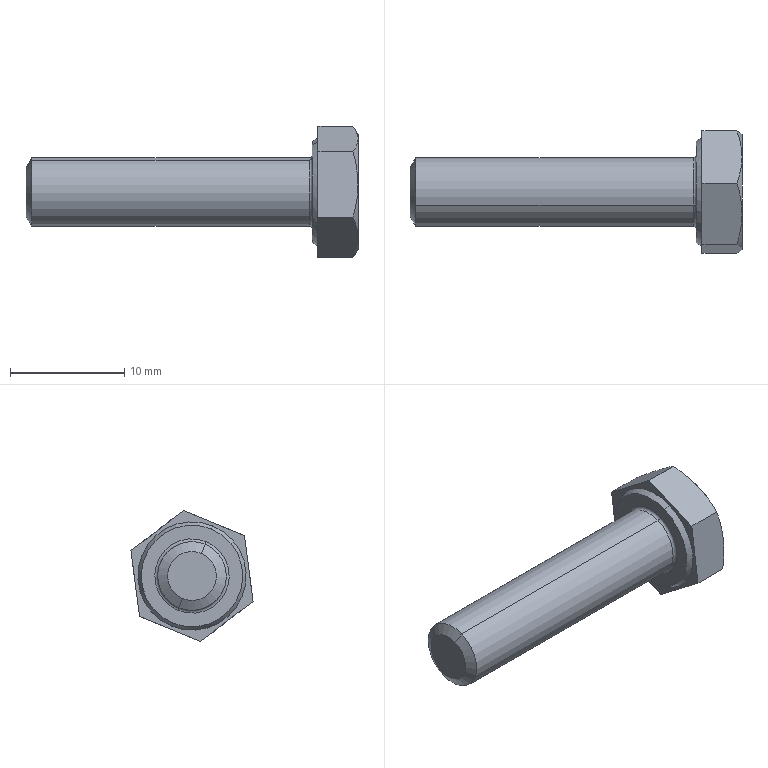Component | NX | HEX_BOLT_M6X25_FT | 1 solid | 24 faces | volume 1038 mm3 | cone 10 | plane 10 | torus 2 | cylinder 2 | commonest cylinder face diameters 6 x2